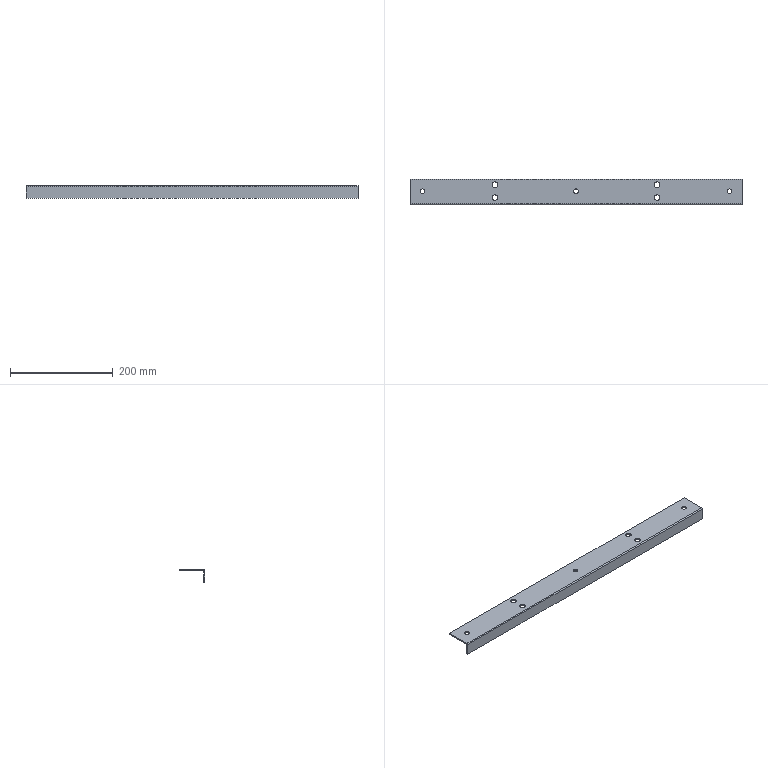Component | SolidWorks | FrameAssembly-1_FrameWeldment-1_UpperBendPlate-1 | 1 solid | 23 faces | box 645 x 50 x 25 mm | volume 114925 mm3 | cylinder 15 | plane 8 | commonest cylinder face diameters 11 x8 9 x6 4 x1
STEP:
#1=COLOUR_RGB('',0.7922,0.8196,0.9333);
#2=FILL_AREA_STYLE_COLOUR('',#1);
#3=FILL_AREA_STYLE('',(#2));
#4=SURFACE_STYLE_FILL_AREA(#3);
#5=SURFACE_SIDE_STYLE('',(#4));
#6=SURFACE_STYLE_USAGE(.BOTH.,#5);
#7=PRESENTATION_STYLE_ASSIGNMENT((#6));
#8=CARTESIAN_POINT('',(-11.939,11.727,-1.339));
#9=VERTEX_POINT('',#8);
#10=CARTESIAN_POINT('',(-11.585,11.727,-1.339));
#11=VERTEX_POINT('',#10);
#12=CARTESIAN_POINT('',(-11.762,11.727,-1.339));
#13=DIRECTION('',(0.,0.,1.));
#14=DIRECTION('',(1.,0.,0.));
#15=AXIS2_PLACEMENT_3D('',#12,#13,#14);
#16=CIRCLE('',#15,0.1772);
#17=EDGE_CURVE('',#9,#11,#16,.T.);
#18=ORIENTED_EDGE('',*,*,#17,.F.);
#19=CARTESIAN_POINT('',(-11.939,11.727,-1.24));
#20=VERTEX_POINT('',#19);
#21=CARTESIAN_POINT('',(-11.939,11.727,-1.24));
#22=DIRECTION('',(0.,0.,1.));
#23=VECTOR('',#22,39.37);
#24=LINE('',#21,#23);
#25=EDGE_CURVE('',#9,#20,#24,.T.);
#26=ORIENTED_EDGE('',*,*,#25,.T.);
#27=CARTESIAN_POINT('',(-11.585,11.727,-1.24));
#28=VERTEX_POINT('',#27);
#29=CARTESIAN_POINT('',(-11.762,11.727,-1.24));
#30=DIRECTION('',(0.,0.,1.));
#31=DIRECTION('',(1.,0.,0.));
#32=AXIS2_PLACEMENT_3D('',#29,#30,#31);
#33=CIRCLE('',#32,0.1772);
#34=EDGE_CURVE('',#20,#28,#33,.T.);
#35=ORIENTED_EDGE('',*,*,#34,.T.);
#36=CARTESIAN_POINT('',(-11.585,11.727,-1.24));
#37=DIRECTION('',(0.,0.,1.));
#38=VECTOR('',#37,39.37);
#39=LINE('',#36,#38);
#40=EDGE_CURVE('',#11,#28,#39,.T.);
#41=ORIENTED_EDGE('',*,*,#40,.F.);
#42=EDGE_LOOP('',(#18,#26,#35,#41));
#43=FACE_OUTER_BOUND('',#42,.T.);
#44=CARTESIAN_POINT('',(-11.762,11.727,-1.24));
#45=DIRECTION('',(0.,0.,1.));
#46=DIRECTION('',(1.,0.,0.));
#47=AXIS2_PLACEMENT_3D('',#44,#45,#46);
#48=CYLINDRICAL_SURFACE('',#47,0.1772);
#49=ADVANCED_FACE('',(#43),#48,.F.);
#50=CARTESIAN_POINT('',(-0.2065,11.727,-1.339));
#51=VERTEX_POINT('',#50);
#52=CARTESIAN_POINT('',(0.1478,11.727,-1.339));
#53=VERTEX_POINT('',#52);
#54=CARTESIAN_POINT('',(-0.02938,11.727,-1.339));
#55=DIRECTION('',(0.,0.,1.));
#56=DIRECTION('',(1.,0.,0.));
#57=AXIS2_PLACEMENT_3D('',#54,#55,#56);
#58=CIRCLE('',#57,0.1772);
#59=EDGE_CURVE('',#51,#53,#58,.T.);
#60=ORIENTED_EDGE('',*,*,#59,.F.);
#61=CARTESIAN_POINT('',(-0.2065,11.727,-1.24));
#62=VERTEX_POINT('',#61);
#63=CARTESIAN_POINT('',(-0.2065,11.727,-1.24));
#64=DIRECTION('',(0.,0.,1.));
#65=VECTOR('',#64,39.37);
#66=LINE('',#63,#65);
#67=EDGE_CURVE('',#51,#62,#66,.T.);
#68=ORIENTED_EDGE('',*,*,#67,.T.);
#69=CARTESIAN_POINT('',(0.1478,11.727,-1.24));
#70=VERTEX_POINT('',#69);
#71=CARTESIAN_POINT('',(-0.02938,11.727,-1.24));
#72=DIRECTION('',(0.,0.,1.));
#73=DIRECTION('',(1.,0.,0.));
#74=AXIS2_PLACEMENT_3D('',#71,#72,#73);
#75=CIRCLE('',#74,0.1772);
#76=EDGE_CURVE('',#62,#70,#75,.T.);
#77=ORIENTED_EDGE('',*,*,#76,.T.);
#78=CARTESIAN_POINT('',(0.1478,11.727,-1.24));
#79=DIRECTION('',(0.,0.,1.));
#80=VECTOR('',#79,39.37);
#81=LINE('',#78,#80);
#82=EDGE_CURVE('',#53,#70,#81,.T.);
#83=ORIENTED_EDGE('',*,*,#82,.F.);
#84=EDGE_LOOP('',(#60,#68,#77,#83));
#85=FACE_OUTER_BOUND('',#84,.T.);
#86=CARTESIAN_POINT('',(-0.02938,11.727,-1.24));
#87=DIRECTION('',(0.,0.,1.));
#88=DIRECTION('',(1.,0.,0.));
#89=AXIS2_PLACEMENT_3D('',#86,#87,#88);
#90=CYLINDRICAL_SURFACE('',#89,0.1772);
#91=ADVANCED_FACE('',(#85),#90,.F.);
#92=CARTESIAN_POINT('',(-23.671,11.727,-1.339));
#93=VERTEX_POINT('',#92);
#94=CARTESIAN_POINT('',(-23.317,11.727,-1.339));
#95=VERTEX_POINT('',#94);
#96=CARTESIAN_POINT('',(-23.494,11.727,-1.339));
#97=DIRECTION('',(0.,0.,1.));
#98=DIRECTION('',(1.,0.,0.));
#99=AXIS2_PLACEMENT_3D('',#96,#97,#98);
#100=CIRCLE('',#99,0.1772);
#101=EDGE_CURVE('',#93,#95,#100,.T.);
#102=ORIENTED_EDGE('',*,*,#101,.F.);
#103=CARTESIAN_POINT('',(-23.671,11.727,-1.24));
#104=VERTEX_POINT('',#103);
#105=CARTESIAN_POINT('',(-23.671,11.727,-1.24));
#106=DIRECTION('',(0.,0.,1.));
#107=VECTOR('',#106,39.37);
#108=LINE('',#105,#107);
#109=EDGE_CURVE('',#93,#104,#108,.T.);
#110=ORIENTED_EDGE('',*,*,#109,.T.);
#111=CARTESIAN_POINT('',(-23.317,11.727,-1.24));
#112=VERTEX_POINT('',#111);
#113=CARTESIAN_POINT('',(-23.494,11.727,-1.24));
#114=DIRECTION('',(0.,0.,1.));
#115=DIRECTION('',(1.,0.,0.));
#116=AXIS2_PLACEMENT_3D('',#113,#114,#115);
#117=CIRCLE('',#116,0.1772);
#118=EDGE_CURVE('',#104,#112,#117,.T.);
#119=ORIENTED_EDGE('',*,*,#118,.T.);
#120=CARTESIAN_POINT('',(-23.317,11.727,-1.24));
#121=DIRECTION('',(0.,0.,1.));
#122=VECTOR('',#121,39.37);
#123=LINE('',#120,#122);
#124=EDGE_CURVE('',#95,#112,#123,.T.);
#125=ORIENTED_EDGE('',*,*,#124,.F.);
#126=EDGE_LOOP('',(#102,#110,#119,#125));
#127=FACE_OUTER_BOUND('',#126,.T.);
#128=CARTESIAN_POINT('',(-23.494,11.727,-1.24));
#129=DIRECTION('',(0.,0.,1.));
#130=DIRECTION('',(1.,0.,0.));
#131=AXIS2_PLACEMENT_3D('',#128,#129,#130);
#132=CYLINDRICAL_SURFACE('',#131,0.1772);
#133=ADVANCED_FACE('',(#127),#132,.F.);
#134=CARTESIAN_POINT('',(-5.777,12.219,-1.339));
#135=VERTEX_POINT('',#134);
#136=CARTESIAN_POINT('',(-5.344,12.219,-1.339));
#137=VERTEX_POINT('',#136);
#138=CARTESIAN_POINT('',(-5.561,12.219,-1.339));
#139=DIRECTION('',(0.,0.,1.));
#140=DIRECTION('',(1.,0.,0.));
#141=AXIS2_PLACEMENT_3D('',#138,#139,#140);
#142=CIRCLE('',#141,0.2165);
#143=EDGE_CURVE('',#135,#137,#142,.T.);
#144=ORIENTED_EDGE('',*,*,#143,.F.);
#145=CARTESIAN_POINT('',(-5.777,12.219,-1.24));
#146=VERTEX_POINT('',#145);
#147=CARTESIAN_POINT('',(-5.777,12.219,-1.24));
#148=DIRECTION('',(0.,0.,1.));
#149=VECTOR('',#148,39.37);
#150=LINE('',#147,#149);
#151=EDGE_CURVE('',#135,#146,#150,.T.);
#152=ORIENTED_EDGE('',*,*,#151,.T.);
#153=CARTESIAN_POINT('',(-5.344,12.219,-1.24));
#154=VERTEX_POINT('',#153);
#155=CARTESIAN_POINT('',(-5.561,12.219,-1.24));
#156=DIRECTION('',(0.,0.,1.));
#157=DIRECTION('',(1.,0.,0.));
#158=AXIS2_PLACEMENT_3D('',#155,#156,#157);
#159=CIRCLE('',#158,0.2165);
#160=EDGE_CURVE('',#146,#154,#159,.T.);
#161=ORIENTED_EDGE('',*,*,#160,.T.);
#162=CARTESIAN_POINT('',(-5.344,12.219,-1.24));
#163=DIRECTION('',(0.,0.,1.));
#164=VECTOR('',#163,39.37);
#165=LINE('',#162,#164);
#166=EDGE_CURVE('',#137,#154,#165,.T.);
#167=ORIENTED_EDGE('',*,*,#166,.F.);
#168=EDGE_LOOP('',(#144,#152,#161,#167));
#169=FACE_OUTER_BOUND('',#168,.T.);
#170=CARTESIAN_POINT('',(-5.561,12.219,-1.24));
#171=DIRECTION('',(0.,0.,1.));
#172=DIRECTION('',(1.,0.,0.));
#173=AXIS2_PLACEMENT_3D('',#170,#171,#172);
#174=CYLINDRICAL_SURFACE('',#173,0.2165);
#175=ADVANCED_FACE('',(#169),#174,.F.);
#176=CARTESIAN_POINT('',(-5.777,11.235,-1.339));
#177=VERTEX_POINT('',#176);
#178=CARTESIAN_POINT('',(-5.344,11.235,-1.339));
#179=VERTEX_POINT('',#178);
#180=CARTESIAN_POINT('',(-5.561,11.235,-1.339));
#181=DIRECTION('',(0.,0.,1.));
#182=DIRECTION('',(1.,0.,0.));
#183=AXIS2_PLACEMENT_3D('',#180,#181,#182);
#184=CIRCLE('',#183,0.2165);
#185=EDGE_CURVE('',#177,#179,#184,.T.);
#186=ORIENTED_EDGE('',*,*,#185,.F.);
#187=CARTESIAN_POINT('',(-5.777,11.235,-1.24));
#188=VERTEX_POINT('',#187);
#189=CARTESIAN_POINT('',(-5.777,11.235,-1.24));
#190=DIRECTION('',(0.,0.,1.));
#191=VECTOR('',#190,39.37);
#192=LINE('',#189,#191);
#193=EDGE_CURVE('',#177,#188,#192,.T.);
#194=ORIENTED_EDGE('',*,*,#193,.T.);
#195=CARTESIAN_POINT('',(-5.344,11.235,-1.24));
#196=VERTEX_POINT('',#195);
#197=CARTESIAN_POINT('',(-5.561,11.235,-1.24));
#198=DIRECTION('',(0.,0.,1.));
#199=DIRECTION('',(1.,0.,0.));
#200=AXIS2_PLACEMENT_3D('',#197,#198,#199);
#201=CIRCLE('',#200,0.2165);
#202=EDGE_CURVE('',#188,#196,#201,.T.);
#203=ORIENTED_EDGE('',*,*,#202,.T.);
#204=CARTESIAN_POINT('',(-5.344,11.235,-1.24));
#205=DIRECTION('',(0.,0.,1.));
#206=VECTOR('',#205,39.37);
#207=LINE('',#204,#206);
#208=EDGE_CURVE('',#179,#196,#207,.T.);
#209=ORIENTED_EDGE('',*,*,#208,.F.);
#210=EDGE_LOOP('',(#186,#194,#203,#209));
#211=FACE_OUTER_BOUND('',#210,.T.);
#212=CARTESIAN_POINT('',(-5.561,11.235,-1.24));
#213=DIRECTION('',(0.,0.,1.));
#214=DIRECTION('',(1.,0.,0.));
#215=AXIS2_PLACEMENT_3D('',#212,#213,#214);
#216=CYLINDRICAL_SURFACE('',#215,0.2165);
#217=ADVANCED_FACE('',(#211),#216,.F.);
#218=CARTESIAN_POINT('',(-18.179,12.219,-1.339));
#219=VERTEX_POINT('',#218);
#220=CARTESIAN_POINT('',(-17.746,12.219,-1.339));
#221=VERTEX_POINT('',#220);
#222=CARTESIAN_POINT('',(-17.962,12.219,-1.339));
#223=DIRECTION('',(0.,0.,1.));
#224=DIRECTION('',(1.,0.,0.));
#225=AXIS2_PLACEMENT_3D('',#222,#223,#224);
#226=CIRCLE('',#225,0.2165);
#227=EDGE_CURVE('',#219,#221,#226,.T.);
#228=ORIENTED_EDGE('',*,*,#227,.F.);
#229=CARTESIAN_POINT('',(-18.179,12.219,-1.24));
#230=VERTEX_POINT('',#229);
#231=CARTESIAN_POINT('',(-18.179,12.219,-1.24));
#232=DIRECTION('',(0.,0.,1.));
#233=VECTOR('',#232,39.37);
#234=LINE('',#231,#233);
#235=EDGE_CURVE('',#219,#230,#234,.T.);
#236=ORIENTED_EDGE('',*,*,#235,.T.);
#237=CARTESIAN_POINT('',(-17.746,12.219,-1.24));
#238=VERTEX_POINT('',#237);
#239=CARTESIAN_POINT('',(-17.962,12.219,-1.24));
#240=DIRECTION('',(0.,0.,1.));
#241=DIRECTION('',(1.,0.,0.));
#242=AXIS2_PLACEMENT_3D('',#239,#240,#241);
#243=CIRCLE('',#242,0.2165);
#244=EDGE_CURVE('',#230,#238,#243,.T.);
#245=ORIENTED_EDGE('',*,*,#244,.T.);
#246=CARTESIAN_POINT('',(-17.746,12.219,-1.24));
#247=DIRECTION('',(0.,0.,1.));
#248=VECTOR('',#247,39.37);
#249=LINE('',#246,#248);
#250=EDGE_CURVE('',#221,#238,#249,.T.);
#251=ORIENTED_EDGE('',*,*,#250,.F.);
#252=EDGE_LOOP('',(#228,#236,#245,#251));
#253=FACE_OUTER_BOUND('',#252,.T.);
#254=CARTESIAN_POINT('',(-17.962,12.219,-1.24));
#255=DIRECTION('',(0.,0.,1.));
#256=DIRECTION('',(1.,0.,0.));
#257=AXIS2_PLACEMENT_3D('',#254,#255,#256);
#258=CYLINDRICAL_SURFACE('',#257,0.2165);
#259=ADVANCED_FACE('',(#253),#258,.F.);
#260=CARTESIAN_POINT('',(-18.179,11.235,-1.339));
#261=VERTEX_POINT('',#260);
#262=CARTESIAN_POINT('',(-17.746,11.235,-1.339));
#263=VERTEX_POINT('',#262);
#264=CARTESIAN_POINT('',(-17.962,11.235,-1.339));
#265=DIRECTION('',(0.,0.,1.));
#266=DIRECTION('',(1.,0.,0.));
#267=AXIS2_PLACEMENT_3D('',#264,#265,#266);
#268=CIRCLE('',#267,0.2165);
#269=EDGE_CURVE('',#261,#263,#268,.T.);
#270=ORIENTED_EDGE('',*,*,#269,.F.);
#271=CARTESIAN_POINT('',(-18.179,11.235,-1.24));
#272=VERTEX_POINT('',#271);
#273=CARTESIAN_POINT('',(-18.179,11.235,-1.24));
#274=DIRECTION('',(0.,0.,1.));
#275=VECTOR('',#274,39.37);
#276=LINE('',#273,#275);
#277=EDGE_CURVE('',#261,#272,#276,.T.);
#278=ORIENTED_EDGE('',*,*,#277,.T.);
#279=CARTESIAN_POINT('',(-17.746,11.235,-1.24));
#280=VERTEX_POINT('',#279);
#281=CARTESIAN_POINT('',(-17.962,11.235,-1.24));
#282=DIRECTION('',(0.,0.,1.));
#283=DIRECTION('',(1.,0.,0.));
#284=AXIS2_PLACEMENT_3D('',#281,#282,#283);
#285=CIRCLE('',#284,0.2165);
#286=EDGE_CURVE('',#272,#280,#285,.T.);
#287=ORIENTED_EDGE('',*,*,#286,.T.);
#288=CARTESIAN_POINT('',(-17.746,11.235,-1.24));
#289=DIRECTION('',(0.,0.,1.));
#290=VECTOR('',#289,39.37);
#291=LINE('',#288,#290);
#292=EDGE_CURVE('',#263,#280,#291,.T.);
#293=ORIENTED_EDGE('',*,*,#292,.F.);
#294=EDGE_LOOP('',(#270,#278,#287,#293));
#295=FACE_OUTER_BOUND('',#294,.T.);
#296=CARTESIAN_POINT('',(-17.962,11.235,-1.24));
#297=DIRECTION('',(0.,0.,1.));
#298=DIRECTION('',(1.,0.,0.));
#299=AXIS2_PLACEMENT_3D('',#296,#297,#298);
#300=CYLINDRICAL_SURFACE('',#299,0.2165);
#301=ADVANCED_FACE('',(#295),#300,.F.);
#302=CARTESIAN_POINT('',(-24.459,10.684,-1.319));
#303=VERTEX_POINT('',#302);
#304=CARTESIAN_POINT('',(-24.459,10.763,-1.24));
#305=VERTEX_POINT('',#304);
#306=CARTESIAN_POINT('',(-24.459,10.763,-1.319));
#307=DIRECTION('',(-1.,-0.,0.));
#308=DIRECTION('',(0.,0.,1.));
#309=AXIS2_PLACEMENT_3D('',#306,#307,#308);
#310=CIRCLE('',#309,0.07874);
#311=EDGE_CURVE('',#303,#305,#310,.T.);
#312=ORIENTED_EDGE('',*,*,#311,.F.);
#313=CARTESIAN_POINT('',(0.9352,10.684,-1.319));
#314=VERTEX_POINT('',#313);
#315=CARTESIAN_POINT('',(0.9352,10.684,-1.319));
#316=DIRECTION('',(-1.,-0.,0.));
#317=VECTOR('',#316,39.37);
#318=LINE('',#315,#317);
#319=EDGE_CURVE('',#314,#303,#318,.T.);
#320=ORIENTED_EDGE('',*,*,#319,.F.);
#321=CARTESIAN_POINT('',(0.9352,10.763,-1.24));
#322=VERTEX_POINT('',#321);
#323=CARTESIAN_POINT('',(0.9352,10.763,-1.319));
#324=DIRECTION('',(-1.,-0.,0.));
#325=DIRECTION('',(0.,0.,1.));
#326=AXIS2_PLACEMENT_3D('',#323,#324,#325);
#327=CIRCLE('',#326,0.07874);
#328=EDGE_CURVE('',#314,#322,#327,.T.);
#329=ORIENTED_EDGE('',*,*,#328,.T.);
#330=CARTESIAN_POINT('',(0.9352,10.763,-1.24));
#331=DIRECTION('',(-1.,-0.,0.));
#332=VECTOR('',#331,39.37);
#333=LINE('',#330,#332);
#334=EDGE_CURVE('',#322,#305,#333,.T.);
#335=ORIENTED_EDGE('',*,*,#334,.T.);
#336=EDGE_LOOP('',(#312,#320,#329,#335));
#337=FACE_OUTER_BOUND('',#336,.T.);
#338=CARTESIAN_POINT('',(0.9352,10.763,-1.319));
#339=DIRECTION('',(-1.,-0.,0.));
#340=DIRECTION('',(0.,0.,1.));
#341=AXIS2_PLACEMENT_3D('',#338,#339,#340);
#342=CYLINDRICAL_SURFACE('',#341,0.07874);
#343=ADVANCED_FACE('',(#337),#342,.T.);
#344=CARTESIAN_POINT('',(-24.459,10.684,-2.224));
#345=VERTEX_POINT('',#344);
#346=CARTESIAN_POINT('',(-24.459,10.684,-2.224));
#347=DIRECTION('',(0.,0.,1.));
#348=VECTOR('',#347,39.37);
#349=LINE('',#346,#348);
#350=EDGE_CURVE('',#345,#303,#349,.T.);
#351=ORIENTED_EDGE('',*,*,#350,.F.);
#352=CARTESIAN_POINT('',(0.9352,10.684,-2.224));
#353=VERTEX_POINT('',#352);
#354=CARTESIAN_POINT('',(0.9352,10.684,-2.224));
#355=DIRECTION('',(-1.,-0.,0.));
#356=VECTOR('',#355,39.37);
#357=LINE('',#354,#356);
#358=EDGE_CURVE('',#353,#345,#357,.T.);
#359=ORIENTED_EDGE('',*,*,#358,.F.);
#360=CARTESIAN_POINT('',(0.9352,10.684,-2.224));
#361=DIRECTION('',(0.,0.,1.));
#362=VECTOR('',#361,39.37);
#363=LINE('',#360,#362);
#364=EDGE_CURVE('',#353,#314,#363,.T.);
#365=ORIENTED_EDGE('',*,*,#364,.T.);
#366=ORIENTED_EDGE('',*,*,#319,.T.);
#367=EDGE_LOOP('',(#351,#359,#365,#366));
#368=FACE_OUTER_BOUND('',#367,.T.);
#369=CARTESIAN_POINT('',(0.9352,10.684,-2.224));
#370=DIRECTION('',(0.,-1.,0.));
#371=DIRECTION('',(-1.,-0.,0.));
#372=AXIS2_PLACEMENT_3D('',#369,#370,#371);
#373=PLANE('',#372);
#374=ADVANCED_FACE('',(#368),#373,.T.);
#375=CARTESIAN_POINT('',(-24.459,10.782,-2.224));
#376=VERTEX_POINT('',#375);
#377=CARTESIAN_POINT('',(0.9352,10.782,-2.224));
#378=VERTEX_POINT('',#377);
#379=CARTESIAN_POINT('',(-24.459,10.782,-2.224));
#380=DIRECTION('',(1.,0.,-0.));
#381=VECTOR('',#380,39.37);
#382=LINE('',#379,#381);
#383=EDGE_CURVE('',#376,#378,#382,.T.);
#384=ORIENTED_EDGE('',*,*,#383,.T.);
#385=CARTESIAN_POINT('',(0.9352,12.652,-2.224));
#386=DIRECTION('',(0.,-1.,0.));
#387=VECTOR('',#386,39.37);
#388=LINE('',#385,#387);
#389=EDGE_CURVE('',#378,#353,#388,.T.);
#390=ORIENTED_EDGE('',*,*,#389,.T.);
#391=ORIENTED_EDGE('',*,*,#358,.T.);
#392=CARTESIAN_POINT('',(-24.459,12.652,-2.224));
#393=DIRECTION('',(0.,-1.,0.));
#394=VECTOR('',#393,39.37);
#395=LINE('',#392,#394);
#396=EDGE_CURVE('',#376,#345,#395,.T.);
#397=ORIENTED_EDGE('',*,*,#396,.F.);
#398=EDGE_LOOP('',(#384,#390,#391,#397));
#399=FACE_OUTER_BOUND('',#398,.T.);
#400=CARTESIAN_POINT('',(0.9352,12.652,-2.224));
#401=DIRECTION('',(-0.,-0.,-1.));
#402=DIRECTION('',(-1.,-0.,0.));
#403=AXIS2_PLACEMENT_3D('',#400,#401,#402);
#404=PLANE('',#403);
#405=ADVANCED_FACE('',(#399),#404,.T.);
#406=CARTESIAN_POINT('',(-24.459,12.652,-1.339));
#407=VERTEX_POINT('',#406);
#408=CARTESIAN_POINT('',(0.9352,12.652,-1.339));
#409=VERTEX_POINT('',#408);
#410=CARTESIAN_POINT('',(-24.459,12.652,-1.339));
#411=DIRECTION('',(1.,0.,-0.));
#412=VECTOR('',#411,39.37);
#413=LINE('',#410,#412);
#414=EDGE_CURVE('',#407,#409,#413,.T.);
#415=ORIENTED_EDGE('',*,*,#414,.F.);
#416=CARTESIAN_POINT('',(-24.459,12.652,-1.24));
#417=VERTEX_POINT('',#416);
#418=CARTESIAN_POINT('',(-24.459,12.652,-1.24));
#419=DIRECTION('',(-0.,-0.,-1.));
#420=VECTOR('',#419,39.37);
#421=LINE('',#418,#420);
#422=EDGE_CURVE('',#417,#407,#421,.T.);
#423=ORIENTED_EDGE('',*,*,#422,.F.);
#424=CARTESIAN_POINT('',(0.9352,12.652,-1.24));
#425=VERTEX_POINT('',#424);
#426=CARTESIAN_POINT('',(0.9352,12.652,-1.24));
#427=DIRECTION('',(-1.,-0.,0.));
#428=VECTOR('',#427,39.37);
#429=LINE('',#426,#428);
#430=EDGE_CURVE('',#425,#417,#429,.T.);
#431=ORIENTED_EDGE('',*,*,#430,.F.);
#432=CARTESIAN_POINT('',(0.9352,12.652,-1.24));
#433=DIRECTION('',(-0.,-0.,-1.));
#434=VECTOR('',#433,39.37);
#435=LINE('',#432,#434);
#436=EDGE_CURVE('',#425,#409,#435,.T.);
#437=ORIENTED_EDGE('',*,*,#436,.T.);
#438=EDGE_LOOP('',(#415,#423,#431,#437));
#439=FACE_OUTER_BOUND('',#438,.T.);
#440=CARTESIAN_POINT('',(0.9352,12.652,-1.24));
#441=DIRECTION('',(-0.,1.,-0.));
#442=DIRECTION('',(1.,0.,-0.));
#443=AXIS2_PLACEMENT_3D('',#440,#441,#442);
#444=PLANE('',#443);
#445=ADVANCED_FACE('',(#439),#444,.T.);
#446=CARTESIAN_POINT('',(-11.762,11.727,-1.24));
#447=DIRECTION('',(0.,0.,1.));
#448=DIRECTION('',(1.,0.,0.));
#449=AXIS2_PLACEMENT_3D('',#446,#447,#448);
#450=CIRCLE('',#449,0.1772);
#451=EDGE_CURVE('',#28,#20,#450,.T.);
#452=ORIENTED_EDGE('',*,*,#451,.F.);
#453=ORIENTED_EDGE('',*,*,#34,.F.);
#454=EDGE_LOOP('',(#452,#453));
#455=FACE_BOUND('',#454,.T.);
#456=CARTESIAN_POINT('',(-0.02938,11.727,-1.24));
#457=DIRECTION('',(0.,0.,1.));
#458=DIRECTION('',(1.,0.,0.));
#459=AXIS2_PLACEMENT_3D('',#456,#457,#458);
#460=CIRCLE('',#459,0.1772);
#461=EDGE_CURVE('',#70,#62,#460,.T.);
#462=ORIENTED_EDGE('',*,*,#461,.F.);
#463=ORIENTED_EDGE('',*,*,#76,.F.);
#464=EDGE_LOOP('',(#462,#463));
#465=FACE_BOUND('',#464,.T.);
#466=CARTESIAN_POINT('',(-23.494,11.727,-1.24));
#467=DIRECTION('',(0.,0.,1.));
#468=DIRECTION('',(1.,0.,0.));
#469=AXIS2_PLACEMENT_3D('',#466,#467,#468);
#470=CIRCLE('',#469,0.1772);
#471=EDGE_CURVE('',#112,#104,#470,.T.);
#472=ORIENTED_EDGE('',*,*,#471,.F.);
#473=ORIENTED_EDGE('',*,*,#118,.F.);
#474=EDGE_LOOP('',(#472,#473));
#475=FACE_BOUND('',#474,.T.);
#476=CARTESIAN_POINT('',(-5.561,12.219,-1.24));
#477=DIRECTION('',(0.,0.,1.));
#478=DIRECTION('',(1.,0.,0.));
#479=AXIS2_PLACEMENT_3D('',#476,#477,#478);
#480=CIRCLE('',#479,0.2165);
#481=EDGE_CURVE('',#154,#146,#480,.T.);
#482=ORIENTED_EDGE('',*,*,#481,.F.);
#483=ORIENTED_EDGE('',*,*,#160,.F.);
#484=EDGE_LOOP('',(#482,#483));
#485=FACE_BOUND('',#484,.T.);
#486=CARTESIAN_POINT('',(-5.561,11.235,-1.24));
#487=DIRECTION('',(0.,0.,1.));
#488=DIRECTION('',(1.,0.,0.));
#489=AXIS2_PLACEMENT_3D('',#486,#487,#488);
#490=CIRCLE('',#489,0.2165);
#491=EDGE_CURVE('',#196,#188,#490,.T.);
#492=ORIENTED_EDGE('',*,*,#491,.F.);
#493=ORIENTED_EDGE('',*,*,#202,.F.);
#494=EDGE_LOOP('',(#492,#493));
#495=FACE_BOUND('',#494,.T.);
#496=CARTESIAN_POINT('',(-17.962,12.219,-1.24));
#497=DIRECTION('',(0.,0.,1.));
#498=DIRECTION('',(1.,0.,0.));
#499=AXIS2_PLACEMENT_3D('',#496,#497,#498);
#500=CIRCLE('',#499,0.2165);
#501=EDGE_CURVE('',#238,#230,#500,.T.);
#502=ORIENTED_EDGE('',*,*,#501,.F.);
#503=ORIENTED_EDGE('',*,*,#244,.F.);
#504=EDGE_LOOP('',(#502,#503));
#505=FACE_BOUND('',#504,.T.);
#506=CARTESIAN_POINT('',(-17.962,11.235,-1.24));
#507=DIRECTION('',(0.,0.,1.));
#508=DIRECTION('',(1.,0.,0.));
#509=AXIS2_PLACEMENT_3D('',#506,#507,#508);
#510=CIRCLE('',#509,0.2165);
#511=EDGE_CURVE('',#280,#272,#510,.T.);
#512=ORIENTED_EDGE('',*,*,#511,.F.);
#513=ORIENTED_EDGE('',*,*,#286,.F.);
#514=EDGE_LOOP('',(#512,#513));
#515=FACE_BOUND('',#514,.T.);
#516=CARTESIAN_POINT('',(-24.459,10.763,-1.24));
#517=DIRECTION('',(-0.,1.,0.));
#518=VECTOR('',#517,39.37);
#519=LINE('',#516,#518);
#520=EDGE_CURVE('',#305,#417,#519,.T.);
#521=ORIENTED_EDGE('',*,*,#520,.F.);
#522=ORIENTED_EDGE('',*,*,#334,.F.);
#523=CARTESIAN_POINT('',(0.9352,10.763,-1.24));
#524=DIRECTION('',(-0.,1.,0.));
#525=VECTOR('',#524,39.37);
#526=LINE('',#523,#525);
#527=EDGE_CURVE('',#322,#425,#526,.T.);
#528=ORIENTED_EDGE('',*,*,#527,.T.);
#529=ORIENTED_EDGE('',*,*,#430,.T.);
#530=EDGE_LOOP('',(#521,#522,#528,#529));
#531=FACE_OUTER_BOUND('',#530,.T.);
#532=CARTESIAN_POINT('',(0.9352,10.763,-1.24));
#533=DIRECTION('',(0.,-0.,1.));
#534=DIRECTION('',(0.,-1.,-0.));
#535=AXIS2_PLACEMENT_3D('',#532,#533,#534);
#536=PLANE('',#535);
#537=ADVANCED_FACE('',(#455,#465,#475,#485,#495,#505,#515,#531),#536,.T.);
#538=CARTESIAN_POINT('',(0.9352,10.782,-1.339));
#539=VERTEX_POINT('',#538);
#540=CARTESIAN_POINT('',(0.9352,10.782,-1.339));
#541=DIRECTION('',(-0.,-0.,-1.));
#542=VECTOR('',#541,39.37);
#543=LINE('',#540,#542);
#544=EDGE_CURVE('',#539,#378,#543,.T.);
#545=ORIENTED_EDGE('',*,*,#544,.F.);
#546=CARTESIAN_POINT('',(0.9352,12.652,-1.339));
#547=DIRECTION('',(0.,-1.,0.));
#548=VECTOR('',#547,39.37);
#549=LINE('',#546,#548);
#550=EDGE_CURVE('',#409,#539,#549,.T.);
#551=ORIENTED_EDGE('',*,*,#550,.F.);
#552=ORIENTED_EDGE('',*,*,#436,.F.);
#553=ORIENTED_EDGE('',*,*,#527,.F.);
#554=ORIENTED_EDGE('',*,*,#328,.F.);
#555=ORIENTED_EDGE('',*,*,#364,.F.);
#556=ORIENTED_EDGE('',*,*,#389,.F.);
#557=EDGE_LOOP('',(#545,#551,#552,#553,#554,#555,#556));
#558=FACE_OUTER_BOUND('',#557,.T.);
#559=CARTESIAN_POINT('',(0.9352,10.763,-1.319));
#560=DIRECTION('',(-1.,-0.,0.));
#561=DIRECTION('',(0.,0.,1.));
#562=AXIS2_PLACEMENT_3D('',#559,#560,#561);
#563=PLANE('',#562);
#564=ADVANCED_FACE('',(#558),#563,.F.);
#565=CARTESIAN_POINT('',(-24.459,10.782,-1.339));
#566=VERTEX_POINT('',#565);
#567=CARTESIAN_POINT('',(-24.459,12.652,-1.339));
#568=DIRECTION('',(0.,-1.,0.));
#569=VECTOR('',#568,39.37);
#570=LINE('',#567,#569);
#571=EDGE_CURVE('',#407,#566,#570,.T.);
#572=ORIENTED_EDGE('',*,*,#571,.T.);
#573=CARTESIAN_POINT('',(-24.459,10.782,-1.339));
#574=DIRECTION('',(-0.,-0.,-1.));
#575=VECTOR('',#574,39.37);
#576=LINE('',#573,#575);
#577=EDGE_CURVE('',#566,#376,#576,.T.);
#578=ORIENTED_EDGE('',*,*,#577,.T.);
#579=ORIENTED_EDGE('',*,*,#396,.T.);
#580=ORIENTED_EDGE('',*,*,#350,.T.);
#581=ORIENTED_EDGE('',*,*,#311,.T.);
#582=ORIENTED_EDGE('',*,*,#520,.T.);
#583=ORIENTED_EDGE('',*,*,#422,.T.);
#584=EDGE_LOOP('',(#572,#578,#579,#580,#581,#582,#583));
#585=FACE_OUTER_BOUND('',#584,.T.);
#586=CARTESIAN_POINT('',(-24.459,10.763,-1.319));
#587=DIRECTION('',(-1.,-0.,0.));
#588=DIRECTION('',(0.,0.,1.));
#589=AXIS2_PLACEMENT_3D('',#586,#587,#588);
#590=PLANE('',#589);
#591=ADVANCED_FACE('',(#585),#590,.T.);
#592=CARTESIAN_POINT('',(-11.762,11.727,-1.339));
#593=DIRECTION('',(0.,0.,1.));
#594=DIRECTION('',(1.,0.,0.));
#595=AXIS2_PLACEMENT_3D('',#592,#593,#594);
#596=CIRCLE('',#595,0.1772);
#597=EDGE_CURVE('',#11,#9,#596,.T.);
#598=ORIENTED_EDGE('',*,*,#597,.T.);
#599=ORIENTED_EDGE('',*,*,#17,.T.);
#600=EDGE_LOOP('',(#598,#599));
#601=FACE_BOUND('',#600,.T.);
#602=CARTESIAN_POINT('',(-0.02938,11.727,-1.339));
#603=DIRECTION('',(0.,0.,1.));
#604=DIRECTION('',(1.,0.,0.));
#605=AXIS2_PLACEMENT_3D('',#602,#603,#604);
#606=CIRCLE('',#605,0.1772);
#607=EDGE_CURVE('',#53,#51,#606,.T.);
#608=ORIENTED_EDGE('',*,*,#607,.T.);
#609=ORIENTED_EDGE('',*,*,#59,.T.);
#610=EDGE_LOOP('',(#608,#609));
#611=FACE_BOUND('',#610,.T.);
#612=CARTESIAN_POINT('',(-23.494,11.727,-1.339));
#613=DIRECTION('',(0.,0.,1.));
#614=DIRECTION('',(1.,0.,0.));
#615=AXIS2_PLACEMENT_3D('',#612,#613,#614);
#616=CIRCLE('',#615,0.1772);
#617=EDGE_CURVE('',#95,#93,#616,.T.);
#618=ORIENTED_EDGE('',*,*,#617,.T.);
#619=ORIENTED_EDGE('',*,*,#101,.T.);
#620=EDGE_LOOP('',(#618,#619));
#621=FACE_BOUND('',#620,.T.);
#622=CARTESIAN_POINT('',(-5.561,12.219,-1.339));
#623=DIRECTION('',(0.,0.,1.));
#624=DIRECTION('',(1.,0.,0.));
#625=AXIS2_PLACEMENT_3D('',#622,#623,#624);
#626=CIRCLE('',#625,0.2165);
#627=EDGE_CURVE('',#137,#135,#626,.T.);
#628=ORIENTED_EDGE('',*,*,#627,.T.);
#629=ORIENTED_EDGE('',*,*,#143,.T.);
#630=EDGE_LOOP('',(#628,#629));
#631=FACE_BOUND('',#630,.T.);
#632=CARTESIAN_POINT('',(-5.561,11.235,-1.339));
#633=DIRECTION('',(0.,0.,1.));
#634=DIRECTION('',(1.,0.,0.));
#635=AXIS2_PLACEMENT_3D('',#632,#633,#634);
#636=CIRCLE('',#635,0.2165);
#637=EDGE_CURVE('',#179,#177,#636,.T.);
#638=ORIENTED_EDGE('',*,*,#637,.T.);
#639=ORIENTED_EDGE('',*,*,#185,.T.);
#640=EDGE_LOOP('',(#638,#639));
#641=FACE_BOUND('',#640,.T.);
#642=CARTESIAN_POINT('',(-17.962,12.219,-1.339));
#643=DIRECTION('',(0.,0.,1.));
#644=DIRECTION('',(1.,0.,0.));
#645=AXIS2_PLACEMENT_3D('',#642,#643,#644);
#646=CIRCLE('',#645,0.2165);
#647=EDGE_CURVE('',#221,#219,#646,.T.);
#648=ORIENTED_EDGE('',*,*,#647,.T.);
#649=ORIENTED_EDGE('',*,*,#227,.T.);
#650=EDGE_LOOP('',(#648,#649));
#651=FACE_BOUND('',#650,.T.);
#652=CARTESIAN_POINT('',(-17.962,11.235,-1.339));
#653=DIRECTION('',(0.,0.,1.));
#654=DIRECTION('',(1.,0.,0.));
#655=AXIS2_PLACEMENT_3D('',#652,#653,#654);
#656=CIRCLE('',#655,0.2165);
#657=EDGE_CURVE('',#263,#261,#656,.T.);
#658=ORIENTED_EDGE('',*,*,#657,.T.);
#659=ORIENTED_EDGE('',*,*,#269,.T.);
#660=EDGE_LOOP('',(#658,#659));
#661=FACE_BOUND('',#660,.T.);
#662=ORIENTED_EDGE('',*,*,#550,.T.);
#663=CARTESIAN_POINT('',(-24.459,10.782,-1.339));
#664=DIRECTION('',(1.,0.,-0.));
#665=VECTOR('',#664,39.37);
#666=LINE('',#663,#665);
#667=EDGE_CURVE('',#566,#539,#666,.T.);
#668=ORIENTED_EDGE('',*,*,#667,.F.);
#669=ORIENTED_EDGE('',*,*,#571,.F.);
#670=ORIENTED_EDGE('',*,*,#414,.T.);
#671=EDGE_LOOP('',(#662,#668,#669,#670));
#672=FACE_OUTER_BOUND('',#671,.T.);
#673=CARTESIAN_POINT('',(-24.459,12.652,-1.339));
#674=DIRECTION('',(0.,0.,1.));
#675=DIRECTION('',(1.,0.,-0.));
#676=AXIS2_PLACEMENT_3D('',#673,#674,#675);
#677=PLANE('',#676);
#678=ADVANCED_FACE('',(#601,#611,#621,#631,#641,#651,#661,#672),#677,.F.);
#679=ORIENTED_EDGE('',*,*,#544,.T.);
#680=ORIENTED_EDGE('',*,*,#383,.F.);
#681=ORIENTED_EDGE('',*,*,#577,.F.);
#682=ORIENTED_EDGE('',*,*,#667,.T.);
#683=EDGE_LOOP('',(#679,#680,#681,#682));
#684=FACE_OUTER_BOUND('',#683,.T.);
#685=CARTESIAN_POINT('',(-24.459,10.782,-1.339));
#686=DIRECTION('',(0.,-1.,0.));
#687=DIRECTION('',(-1.,-0.,0.));
#688=AXIS2_PLACEMENT_3D('',#685,#686,#687);
#689=PLANE('',#688);
#690=ADVANCED_FACE('',(#684),#689,.F.);
#691=ORIENTED_EDGE('',*,*,#277,.F.);
#692=ORIENTED_EDGE('',*,*,#657,.F.);
#693=ORIENTED_EDGE('',*,*,#292,.T.);
#694=ORIENTED_EDGE('',*,*,#511,.T.);
#695=EDGE_LOOP('',(#691,#692,#693,#694));
#696=FACE_OUTER_BOUND('',#695,.T.);
#697=CARTESIAN_POINT('',(-17.962,11.235,-1.24));
#698=DIRECTION('',(0.,0.,1.));
#699=DIRECTION('',(1.,0.,0.));
#700=AXIS2_PLACEMENT_3D('',#697,#698,#699);
#701=CYLINDRICAL_SURFACE('',#700,0.2165);
#702=ADVANCED_FACE('',(#696),#701,.F.);
#703=ORIENTED_EDGE('',*,*,#235,.F.);
#704=ORIENTED_EDGE('',*,*,#647,.F.);
#705=ORIENTED_EDGE('',*,*,#250,.T.);
#706=ORIENTED_EDGE('',*,*,#501,.T.);
#707=EDGE_LOOP('',(#703,#704,#705,#706));
#708=FACE_OUTER_BOUND('',#707,.T.);
#709=CARTESIAN_POINT('',(-17.962,12.219,-1.24));
#710=DIRECTION('',(0.,0.,1.));
#711=DIRECTION('',(1.,0.,0.));
#712=AXIS2_PLACEMENT_3D('',#709,#710,#711);
#713=CYLINDRICAL_SURFACE('',#712,0.2165);
#714=ADVANCED_FACE('',(#708),#713,.F.);
#715=ORIENTED_EDGE('',*,*,#193,.F.);
#716=ORIENTED_EDGE('',*,*,#637,.F.);
#717=ORIENTED_EDGE('',*,*,#208,.T.);
#718=ORIENTED_EDGE('',*,*,#491,.T.);
#719=EDGE_LOOP('',(#715,#716,#717,#718));
#720=FACE_OUTER_BOUND('',#719,.T.);
#721=CARTESIAN_POINT('',(-5.561,11.235,-1.24));
#722=DIRECTION('',(0.,0.,1.));
#723=DIRECTION('',(1.,0.,0.));
#724=AXIS2_PLACEMENT_3D('',#721,#722,#723);
#725=CYLINDRICAL_SURFACE('',#724,0.2165);
#726=ADVANCED_FACE('',(#720),#725,.F.);
#727=ORIENTED_EDGE('',*,*,#151,.F.);
#728=ORIENTED_EDGE('',*,*,#627,.F.);
#729=ORIENTED_EDGE('',*,*,#166,.T.);
#730=ORIENTED_EDGE('',*,*,#481,.T.);
#731=EDGE_LOOP('',(#727,#728,#729,#730));
#732=FACE_OUTER_BOUND('',#731,.T.);
#733=CARTESIAN_POINT('',(-5.561,12.219,-1.24));
#734=DIRECTION('',(0.,0.,1.));
#735=DIRECTION('',(1.,0.,0.));
#736=AXIS2_PLACEMENT_3D('',#733,#734,#735);
#737=CYLINDRICAL_SURFACE('',#736,0.2165);
#738=ADVANCED_FACE('',(#732),#737,.F.);
#739=ORIENTED_EDGE('',*,*,#109,.F.);
#740=ORIENTED_EDGE('',*,*,#617,.F.);
#741=ORIENTED_EDGE('',*,*,#124,.T.);
#742=ORIENTED_EDGE('',*,*,#471,.T.);
#743=EDGE_LOOP('',(#739,#740,#741,#742));
#744=FACE_OUTER_BOUND('',#743,.T.);
#745=CARTESIAN_POINT('',(-23.494,11.727,-1.24));
#746=DIRECTION('',(0.,0.,1.));
#747=DIRECTION('',(1.,0.,0.));
#748=AXIS2_PLACEMENT_3D('',#745,#746,#747);
#749=CYLINDRICAL_SURFACE('',#748,0.1772);
#750=ADVANCED_FACE('',(#744),#749,.F.);
#751=ORIENTED_EDGE('',*,*,#67,.F.);
#752=ORIENTED_EDGE('',*,*,#607,.F.);
#753=ORIENTED_EDGE('',*,*,#82,.T.);
#754=ORIENTED_EDGE('',*,*,#461,.T.);
#755=EDGE_LOOP('',(#751,#752,#753,#754));
#756=FACE_OUTER_BOUND('',#755,.T.);
#757=CARTESIAN_POINT('',(-0.02938,11.727,-1.24));
#758=DIRECTION('',(0.,0.,1.));
#759=DIRECTION('',(1.,0.,0.));
#760=AXIS2_PLACEMENT_3D('',#757,#758,#759);
#761=CYLINDRICAL_SURFACE('',#760,0.1772);
#762=ADVANCED_FACE('',(#756),#761,.F.);
#763=ORIENTED_EDGE('',*,*,#25,.F.);
#764=ORIENTED_EDGE('',*,*,#597,.F.);
#765=ORIENTED_EDGE('',*,*,#40,.T.);
#766=ORIENTED_EDGE('',*,*,#451,.T.);
#767=EDGE_LOOP('',(#763,#764,#765,#766));
#768=FACE_OUTER_BOUND('',#767,.T.);
#769=CARTESIAN_POINT('',(-11.762,11.727,-1.24));
#770=DIRECTION('',(0.,0.,1.));
#771=DIRECTION('',(1.,0.,0.));
#772=AXIS2_PLACEMENT_3D('',#769,#770,#771);
#773=CYLINDRICAL_SURFACE('',#772,0.1772);
#774=ADVANCED_FACE('',(#768),#773,.F.);
#775=CLOSED_SHELL('',(#49,#91,#133,#175,#217,#259,#301,#343,#374,#405,#445,#537,#564,#591,#678,#690,#702,#714,#726,#738,#750,#762,#774));
#776=MANIFOLD_SOLID_BREP('',#775);
#777=STYLED_ITEM('',(#7),#776);
#778=(LENGTH_UNIT()NAMED_UNIT(*)SI_UNIT($,.METRE.));
#779=LENGTH_MEASURE_WITH_UNIT(LENGTH_MEASURE(0.0254),#778);
#780=DIMENSIONAL_EXPONENTS(1.,0.,0.,0.,0.,0.,0.);
#781=(CONVERSION_BASED_UNIT('',#779)LENGTH_UNIT()NAMED_UNIT(#780));
#782=UNCERTAINTY_MEASURE_WITH_UNIT(LENGTH_MEASURE(0.00001),#781,'','');
#783=(NAMED_UNIT(*)PLANE_ANGLE_UNIT()SI_UNIT($,.RADIAN.));
#784=(NAMED_UNIT(*)SI_UNIT($,.STERADIAN.)SOLID_ANGLE_UNIT());
#785=(GEOMETRIC_REPRESENTATION_CONTEXT(3)GLOBAL_UNCERTAINTY_ASSIGNED_CONTEXT((#782))GLOBAL_UNIT_ASSIGNED_CONTEXT((#781,#783,#784))REPRESENTATION_CONTEXT('',''));
#786=MECHANICAL_DESIGN_GEOMETRIC_PRESENTATION_REPRESENTATION('',(#777),#785);
#787=PRESENTATION_LAYER_ASSIGNMENT('','',(#777));
#788=CARTESIAN_POINT('',(0.,0.,0.));
#789=DIRECTION('',(0.,0.,1.));
#790=DIRECTION('',(1.,0.,0.));
#791=AXIS2_PLACEMENT_3D('',#788,#789,#790);
#792=(LENGTH_UNIT()NAMED_UNIT(*)SI_UNIT($,.METRE.));
#793=LENGTH_MEASURE_WITH_UNIT(LENGTH_MEASURE(0.0254),#792);
#794=DIMENSIONAL_EXPONENTS(1.,0.,0.,0.,0.,0.,0.);
#795=(CONVERSION_BASED_UNIT('',#793)LENGTH_UNIT()NAMED_UNIT(#794));
#796=UNCERTAINTY_MEASURE_WITH_UNIT(LENGTH_MEASURE(0.00001),#795,'','');
#797=(NAMED_UNIT(*)PLANE_ANGLE_UNIT()SI_UNIT($,.RADIAN.));
#798=(NAMED_UNIT(*)SI_UNIT($,.STERADIAN.)SOLID_ANGLE_UNIT());
#799=(GEOMETRIC_REPRESENTATION_CONTEXT(3)GLOBAL_UNCERTAINTY_ASSIGNED_CONTEXT((#796))GLOBAL_UNIT_ASSIGNED_CONTEXT((#795,#797,#798))REPRESENTATION_CONTEXT('',''));
#800=ADVANCED_BREP_SHAPE_REPRESENTATION('',(#776,#791),#799);